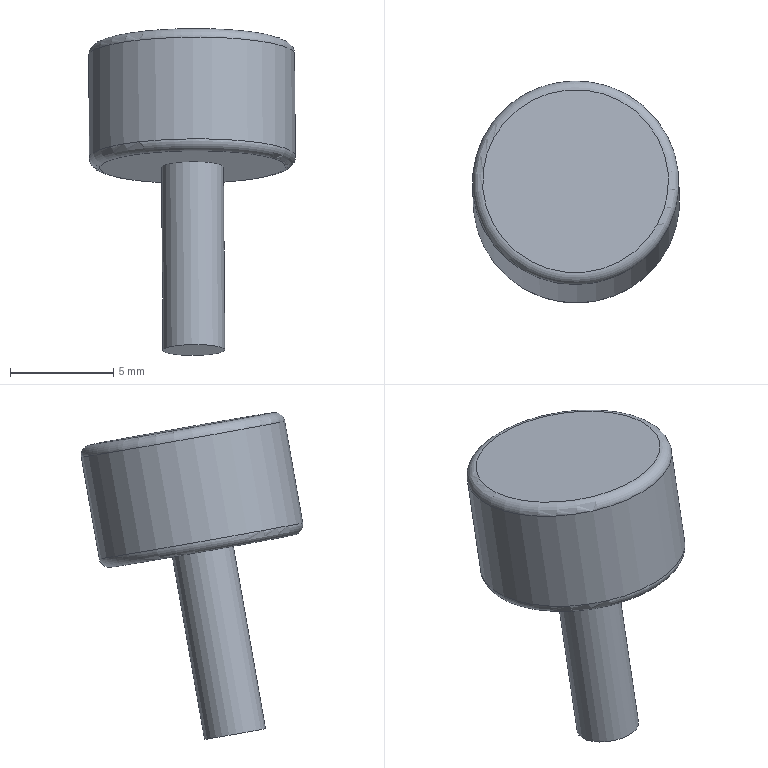Component | NX | 16 | 1 solid | 7 faces | box 10.04 x 10.73 x 15.82 mm | volume 532 mm3 | plane 3 | cylinder 2 | torus 2 | commonest cylinder face diameters 10 x1 3 x1
STEP:
#1=CARTESIAN_POINT('',(0.,0.,0.));
#2=DIRECTION('',(0.,0.,1.));
#3=DIRECTION('',(1.,0.,0.));
#4=AXIS2_PLACEMENT_3D('',#1,#2,#3);
#5=CARTESIAN_POINT('',(88.843,266.854,149.684));
#6=VERTEX_POINT('',#5);
#7=CARTESIAN_POINT('',(84.048,265.455,149.893));
#8=DIRECTION('',(0.00764,-0.1736,-0.9848));
#9=DIRECTION('',(0.9591,0.2798,-0.0419));
#10=AXIS2_PLACEMENT_3D('',#7,#8,#9);
#11=CIRCLE('',#10,5.);
#12=CARTESIAN_POINT('',(84.09,264.5,144.477));
#13=DIRECTION('',(-0.00764,0.1736,0.9848));
#14=DIRECTION('',(-0.9591,-0.2798,0.0419));
#15=AXIS2_PLACEMENT_3D('',#12,#13,#14);
#16=CYLINDRICAL_SURFACE('',#15,5.);
#17=CARTESIAN_POINT('',(9.425,5.5));
#18=DIRECTION('',(-1.,0.));
#19=VECTOR('',#18,1.);
#20=LINE('',#17,#19);
#21=(GEOMETRIC_REPRESENTATION_CONTEXT(2)PARAMETRIC_REPRESENTATION_CONTEXT()REPRESENTATION_CONTEXT('',''));
#22=DEFINITIONAL_REPRESENTATION('',(#20),#21);
#23=PCURVE('',#16,#22);
#24=CARTESIAN_POINT('',(84.048,265.455,149.893));
#25=DIRECTION('',(0.00764,-0.1736,-0.9848));
#26=DIRECTION('',(0.9591,0.2798,-0.0419));
#27=AXIS2_PLACEMENT_3D('',#24,#25,#26);
#28=TOROIDAL_SURFACE('',#27,4.5,0.5);
#29=CARTESIAN_POINT('',(0.,6.283));
#30=DIRECTION('',(1.,0.));
#31=VECTOR('',#30,1.);
#32=LINE('',#29,#31);
#33=(GEOMETRIC_REPRESENTATION_CONTEXT(2)PARAMETRIC_REPRESENTATION_CONTEXT()REPRESENTATION_CONTEXT('',''));
#34=DEFINITIONAL_REPRESENTATION('',(#32),#33);
#35=PCURVE('',#28,#34);
#36=SURFACE_CURVE('',#11,(#23,#35),.PCURVE_S1.);
#37=EDGE_CURVE('',#6,#6,#36,.T.);
#38=ORIENTED_EDGE('',*,*,#37,.T.);
#39=CARTESIAN_POINT('',(88.882,265.986,144.76));
#40=VERTEX_POINT('',#39);
#41=CARTESIAN_POINT('',(88.882,265.986,144.76));
#42=CARTESIAN_POINT('',(88.843,266.854,149.684));
#43=B_SPLINE_CURVE_WITH_KNOTS('',1,(#41,#42),.UNSPECIFIED.,.F.,.F.,(2,2),(0.5,5.5),.PIECEWISE_BEZIER_KNOTS.);
#44=CARTESIAN_POINT('',(3.142,0.));
#45=DIRECTION('',(0.,1.));
#46=VECTOR('',#45,1.);
#47=LINE('',#44,#46);
#48=(GEOMETRIC_REPRESENTATION_CONTEXT(2)PARAMETRIC_REPRESENTATION_CONTEXT()REPRESENTATION_CONTEXT('',''));
#49=DEFINITIONAL_REPRESENTATION('',(#47),#48);
#50=PCURVE('',#16,#49);
#51=CARTESIAN_POINT('',(9.425,0.));
#52=DIRECTION('',(0.,1.));
#53=VECTOR('',#52,1.);
#54=LINE('',#51,#53);
#55=(GEOMETRIC_REPRESENTATION_CONTEXT(2)PARAMETRIC_REPRESENTATION_CONTEXT()REPRESENTATION_CONTEXT('',''));
#56=DEFINITIONAL_REPRESENTATION('',(#54),#55);
#57=PCURVE('',#16,#56);
#58=SEAM_CURVE('',#43,(#50,#57),.PCURVE_S1.);
#59=EDGE_CURVE('',#40,#6,#58,.T.);
#60=ORIENTED_EDGE('',*,*,#59,.F.);
#61=CARTESIAN_POINT('',(84.086,264.586,144.969));
#62=DIRECTION('',(-0.00764,0.1736,0.9848));
#63=DIRECTION('',(0.9591,0.2798,-0.0419));
#64=AXIS2_PLACEMENT_3D('',#61,#62,#63);
#65=CIRCLE('',#64,5.);
#66=CARTESIAN_POINT('',(3.142,0.5));
#67=DIRECTION('',(1.,0.));
#68=VECTOR('',#67,1.);
#69=LINE('',#66,#68);
#70=(GEOMETRIC_REPRESENTATION_CONTEXT(2)PARAMETRIC_REPRESENTATION_CONTEXT()REPRESENTATION_CONTEXT('',''));
#71=DEFINITIONAL_REPRESENTATION('',(#69),#70);
#72=PCURVE('',#16,#71);
#73=CARTESIAN_POINT('',(84.086,264.586,144.969));
#74=DIRECTION('',(0.00764,-0.1736,-0.9848));
#75=DIRECTION('',(0.9591,0.2798,-0.0419));
#76=AXIS2_PLACEMENT_3D('',#73,#74,#75);
#77=TOROIDAL_SURFACE('',#76,4.5,0.5);
#78=CARTESIAN_POINT('',(6.283,6.283));
#79=CARTESIAN_POINT('',(6.188,6.283));
#80=CARTESIAN_POINT('',(5.998,6.283));
#81=CARTESIAN_POINT('',(5.712,6.283));
#82=CARTESIAN_POINT('',(5.426,6.283));
#83=CARTESIAN_POINT('',(5.141,6.283));
#84=CARTESIAN_POINT('',(4.855,6.283));
#85=CARTESIAN_POINT('',(4.57,6.283));
#86=CARTESIAN_POINT('',(4.284,6.283));
#87=CARTESIAN_POINT('',(3.998,6.283));
#88=CARTESIAN_POINT('',(3.713,6.283));
#89=CARTESIAN_POINT('',(3.427,6.283));
#90=CARTESIAN_POINT('',(3.142,6.283));
#91=CARTESIAN_POINT('',(2.856,6.283));
#92=CARTESIAN_POINT('',(2.57,6.283));
#93=CARTESIAN_POINT('',(2.285,6.283));
#94=CARTESIAN_POINT('',(1.999,6.283));
#95=CARTESIAN_POINT('',(1.714,6.283));
#96=CARTESIAN_POINT('',(1.428,6.283));
#97=CARTESIAN_POINT('',(1.142,6.283));
#98=CARTESIAN_POINT('',(0.8568,6.283));
#99=CARTESIAN_POINT('',(0.5712,6.283));
#100=CARTESIAN_POINT('',(0.2856,6.283));
#101=CARTESIAN_POINT('',(0.0952,6.283));
#102=CARTESIAN_POINT('',(0.,6.283));
#103=B_SPLINE_CURVE_WITH_KNOTS('',3,(#78,#79,#80,#81,#82,#83,#84,#85,#86,#87,#88,#89,#90,#91,#92,#93,#94,#95,#96,#97,#98,#99,#100,#101,#102),.UNSPECIFIED.,.F.,.F.,(4,1,1,1,1,1,1,1,1,1,1,1,1,1,1,1,1,1,1,1,1,1,4),(0.,0.2856,0.5712,0.8568,1.142,1.428,1.714,1.999,2.285,2.57,2.856,3.142,3.427,3.713,3.998,4.284,4.57,4.855,5.141,5.426,5.712,5.998,6.283),.QUASI_UNIFORM_KNOTS.);
#104=(GEOMETRIC_REPRESENTATION_CONTEXT(2)PARAMETRIC_REPRESENTATION_CONTEXT()REPRESENTATION_CONTEXT('',''));
#105=DEFINITIONAL_REPRESENTATION('',(#103),#104);
#106=PCURVE('',#77,#105);
#107=SURFACE_CURVE('',#65,(#72,#106),.PCURVE_S1.);
#108=EDGE_CURVE('',#40,#40,#107,.T.);
#109=ORIENTED_EDGE('',*,*,#108,.T.);
#110=ORIENTED_EDGE('',*,*,#59,.T.);
#111=EDGE_LOOP('',(#38,#60,#109,#110));
#112=FACE_BOUND('',#111,.T.);
#113=ADVANCED_FACE('',(#112),#16,.T.);
#114=CARTESIAN_POINT('',(88.406,265.759,144.288));
#115=VERTEX_POINT('',#114);
#116=CARTESIAN_POINT('',(84.09,264.5,144.477));
#117=DIRECTION('',(0.00764,-0.1736,-0.9848));
#118=DIRECTION('',(0.9591,0.2798,-0.0419));
#119=AXIS2_PLACEMENT_3D('',#116,#117,#118);
#120=CIRCLE('',#119,4.5);
#121=CARTESIAN_POINT('',(84.09,264.5,144.477));
#122=DIRECTION('',(0.00764,-0.1736,-0.9848));
#123=DIRECTION('',(0.9591,0.2798,-0.0419));
#124=AXIS2_PLACEMENT_3D('',#121,#122,#123);
#125=PLANE('',#124);
#126=CARTESIAN_POINT('',(0.,0.));
#127=DIRECTION('',(1.,0.));
#128=AXIS2_PLACEMENT_2D('',#126,#127);
#129=CIRCLE('',#128,4.5);
#130=(GEOMETRIC_REPRESENTATION_CONTEXT(2)PARAMETRIC_REPRESENTATION_CONTEXT()REPRESENTATION_CONTEXT('',''));
#131=DEFINITIONAL_REPRESENTATION('',(#129),#130);
#132=PCURVE('',#125,#131);
#133=CARTESIAN_POINT('',(0.,7.854));
#134=DIRECTION('',(1.,0.));
#135=VECTOR('',#134,1.);
#136=LINE('',#133,#135);
#137=(GEOMETRIC_REPRESENTATION_CONTEXT(2)PARAMETRIC_REPRESENTATION_CONTEXT()REPRESENTATION_CONTEXT('',''));
#138=DEFINITIONAL_REPRESENTATION('',(#136),#137);
#139=PCURVE('',#77,#138);
#140=SURFACE_CURVE('',#120,(#132,#139),.PCURVE_S1.);
#141=EDGE_CURVE('',#115,#115,#140,.T.);
#142=ORIENTED_EDGE('',*,*,#141,.T.);
#143=EDGE_LOOP('',(#142));
#144=FACE_BOUND('',#143,.T.);
#145=CARTESIAN_POINT('',(85.528,264.919,144.414));
#146=VERTEX_POINT('',#145);
#147=CARTESIAN_POINT('',(84.09,264.5,144.477));
#148=DIRECTION('',(0.00764,-0.1736,-0.9848));
#149=DIRECTION('',(0.9591,0.2798,-0.0419));
#150=AXIS2_PLACEMENT_3D('',#147,#148,#149);
#151=CIRCLE('',#150,1.5);
#152=CARTESIAN_POINT('',(0.,0.));
#153=DIRECTION('',(1.,-0.));
#154=AXIS2_PLACEMENT_2D('',#152,#153);
#155=CIRCLE('',#154,1.5);
#156=(GEOMETRIC_REPRESENTATION_CONTEXT(2)PARAMETRIC_REPRESENTATION_CONTEXT()REPRESENTATION_CONTEXT('',''));
#157=DEFINITIONAL_REPRESENTATION('',(#155),#156);
#158=PCURVE('',#125,#157);
#159=CARTESIAN_POINT('',(84.159,262.937,135.614));
#160=DIRECTION('',(-0.00764,0.1736,0.9848));
#161=DIRECTION('',(-0.9591,-0.2798,0.0419));
#162=AXIS2_PLACEMENT_3D('',#159,#160,#161);
#163=CYLINDRICAL_SURFACE('',#162,1.5);
#164=CARTESIAN_POINT('',(9.425,9.));
#165=DIRECTION('',(-1.,0.));
#166=VECTOR('',#165,1.);
#167=LINE('',#164,#166);
#168=(GEOMETRIC_REPRESENTATION_CONTEXT(2)PARAMETRIC_REPRESENTATION_CONTEXT()REPRESENTATION_CONTEXT('',''));
#169=DEFINITIONAL_REPRESENTATION('',(#167),#168);
#170=PCURVE('',#163,#169);
#171=SURFACE_CURVE('',#151,(#158,#170),.PCURVE_S1.);
#172=EDGE_CURVE('',#146,#146,#171,.T.);
#173=ORIENTED_EDGE('',*,*,#172,.F.);
#174=EDGE_LOOP('',(#173));
#175=FACE_BOUND('',#174,.T.);
#176=ADVANCED_FACE('',(#144,#175),#125,.T.);
#177=CARTESIAN_POINT('',(88.36,266.801,150.197));
#178=VERTEX_POINT('',#177);
#179=CARTESIAN_POINT('',(84.044,265.542,150.385));
#180=DIRECTION('',(-0.00764,0.1736,0.9848));
#181=DIRECTION('',(0.9591,0.2798,-0.0419));
#182=AXIS2_PLACEMENT_3D('',#179,#180,#181);
#183=CIRCLE('',#182,4.5);
#184=CARTESIAN_POINT('',(84.044,265.542,150.385));
#185=DIRECTION('',(0.00764,-0.1736,-0.9848));
#186=DIRECTION('',(0.9591,0.2798,-0.0419));
#187=AXIS2_PLACEMENT_3D('',#184,#185,#186);
#188=PLANE('',#187);
#189=CARTESIAN_POINT('',(4.5,0.));
#190=CARTESIAN_POINT('',(4.5,-7.794));
#191=CARTESIAN_POINT('',(-2.25,-3.897));
#192=CARTESIAN_POINT('',(-9.,-0.));
#193=CARTESIAN_POINT('',(-2.25,3.897));
#194=CARTESIAN_POINT('',(4.5,7.794));
#195=CARTESIAN_POINT('',(4.5,0.));
#196=(BOUNDED_CURVE()B_SPLINE_CURVE(2,(#189,#190,#191,#192,#193,#194,#195),.UNSPECIFIED.,.T.,.F.)B_SPLINE_CURVE_WITH_KNOTS((1,2,2,2,2,1),(-2.094,0.,2.094,4.189,6.283,8.378),.UNSPECIFIED.)CURVE()GEOMETRIC_REPRESENTATION_ITEM()RATIONAL_B_SPLINE_CURVE((1.,0.5,1.,0.5,1.,0.5,1.))REPRESENTATION_ITEM(''));
#197=(GEOMETRIC_REPRESENTATION_CONTEXT(2)PARAMETRIC_REPRESENTATION_CONTEXT()REPRESENTATION_CONTEXT('',''));
#198=DEFINITIONAL_REPRESENTATION('',(#196),#197);
#199=PCURVE('',#188,#198);
#200=CARTESIAN_POINT('',(6.283,4.712));
#201=DIRECTION('',(-1.,0.));
#202=VECTOR('',#201,1.);
#203=LINE('',#200,#202);
#204=(GEOMETRIC_REPRESENTATION_CONTEXT(2)PARAMETRIC_REPRESENTATION_CONTEXT()REPRESENTATION_CONTEXT('',''));
#205=DEFINITIONAL_REPRESENTATION('',(#203),#204);
#206=PCURVE('',#28,#205);
#207=SURFACE_CURVE('',#183,(#199,#206),.PCURVE_S1.);
#208=EDGE_CURVE('',#178,#178,#207,.T.);
#209=ORIENTED_EDGE('',*,*,#208,.T.);
#210=EDGE_LOOP('',(#209));
#211=FACE_BOUND('',#210,.T.);
#212=ADVANCED_FACE('',(#211),#188,.F.);
#213=CARTESIAN_POINT('',(85.597,263.357,135.551));
#214=VERTEX_POINT('',#213);
#215=CARTESIAN_POINT('',(84.159,262.937,135.614));
#216=DIRECTION('',(0.00764,-0.1736,-0.9848));
#217=DIRECTION('',(0.9591,0.2798,-0.0419));
#218=AXIS2_PLACEMENT_3D('',#215,#216,#217);
#219=CIRCLE('',#218,1.5);
#220=CARTESIAN_POINT('',(9.425,0.));
#221=DIRECTION('',(-1.,0.));
#222=VECTOR('',#221,1.);
#223=LINE('',#220,#222);
#224=(GEOMETRIC_REPRESENTATION_CONTEXT(2)PARAMETRIC_REPRESENTATION_CONTEXT()REPRESENTATION_CONTEXT('',''));
#225=DEFINITIONAL_REPRESENTATION('',(#223),#224);
#226=PCURVE('',#163,#225);
#227=CARTESIAN_POINT('',(84.159,262.937,135.614));
#228=DIRECTION('',(0.00764,-0.1736,-0.9848));
#229=DIRECTION('',(0.9591,0.2798,-0.0419));
#230=AXIS2_PLACEMENT_3D('',#227,#228,#229);
#231=PLANE('',#230);
#232=CARTESIAN_POINT('',(0.,0.));
#233=DIRECTION('',(1.,-0.));
#234=AXIS2_PLACEMENT_2D('',#232,#233);
#235=CIRCLE('',#234,1.5);
#236=(GEOMETRIC_REPRESENTATION_CONTEXT(2)PARAMETRIC_REPRESENTATION_CONTEXT()REPRESENTATION_CONTEXT('',''));
#237=DEFINITIONAL_REPRESENTATION('',(#235),#236);
#238=PCURVE('',#231,#237);
#239=SURFACE_CURVE('',#219,(#226,#238),.PCURVE_S1.);
#240=EDGE_CURVE('',#214,#214,#239,.T.);
#241=ORIENTED_EDGE('',*,*,#240,.F.);
#242=CARTESIAN_POINT('',(85.597,263.357,135.551));
#243=CARTESIAN_POINT('',(85.528,264.919,144.414));
#244=B_SPLINE_CURVE_WITH_KNOTS('',1,(#242,#243),.UNSPECIFIED.,.F.,.F.,(2,2),(0.,9.),.PIECEWISE_BEZIER_KNOTS.);
#245=CARTESIAN_POINT('',(9.425,0.));
#246=DIRECTION('',(0.,1.));
#247=VECTOR('',#246,1.);
#248=LINE('',#245,#247);
#249=(GEOMETRIC_REPRESENTATION_CONTEXT(2)PARAMETRIC_REPRESENTATION_CONTEXT()REPRESENTATION_CONTEXT('',''));
#250=DEFINITIONAL_REPRESENTATION('',(#248),#249);
#251=PCURVE('',#163,#250);
#252=CARTESIAN_POINT('',(3.142,0.));
#253=DIRECTION('',(0.,1.));
#254=VECTOR('',#253,1.);
#255=LINE('',#252,#254);
#256=(GEOMETRIC_REPRESENTATION_CONTEXT(2)PARAMETRIC_REPRESENTATION_CONTEXT()REPRESENTATION_CONTEXT('',''));
#257=DEFINITIONAL_REPRESENTATION('',(#255),#256);
#258=PCURVE('',#163,#257);
#259=SEAM_CURVE('',#244,(#251,#258),.PCURVE_S1.);
#260=EDGE_CURVE('',#214,#146,#259,.T.);
#261=ORIENTED_EDGE('',*,*,#260,.T.);
#262=ORIENTED_EDGE('',*,*,#172,.T.);
#263=ORIENTED_EDGE('',*,*,#260,.F.);
#264=EDGE_LOOP('',(#241,#261,#262,#263));
#265=FACE_BOUND('',#264,.T.);
#266=ADVANCED_FACE('',(#265),#163,.T.);
#267=ORIENTED_EDGE('',*,*,#240,.T.);
#268=EDGE_LOOP('',(#267));
#269=FACE_BOUND('',#268,.T.);
#270=ADVANCED_FACE('',(#269),#231,.T.);
#271=ORIENTED_EDGE('',*,*,#208,.F.);
#272=CARTESIAN_POINT('',(88.36,266.801,150.197));
#273=CARTESIAN_POINT('',(88.488,266.838,150.191));
#274=CARTESIAN_POINT('',(88.613,266.867,150.144));
#275=CARTESIAN_POINT('',(88.722,266.884,150.059));
#276=CARTESIAN_POINT('',(88.801,266.888,149.945));
#277=CARTESIAN_POINT('',(88.842,266.877,149.815));
#278=CARTESIAN_POINT('',(88.843,266.854,149.684));
#279=(BOUNDED_CURVE()B_SPLINE_CURVE(6,(#272,#273,#274,#275,#276,#277,#278),.UNSPECIFIED.,.F.,.F.)B_SPLINE_CURVE_WITH_KNOTS((7,7),(4.712,6.283),.PIECEWISE_BEZIER_KNOTS.)CURVE()GEOMETRIC_REPRESENTATION_ITEM()RATIONAL_B_SPLINE_CURVE((1.031,1.01,0.9979,0.994,0.9979,1.01,1.031))REPRESENTATION_ITEM(''));
#280=CARTESIAN_POINT('',(6.283,0.));
#281=DIRECTION('',(0.,1.));
#282=VECTOR('',#281,1.);
#283=LINE('',#280,#282);
#284=(GEOMETRIC_REPRESENTATION_CONTEXT(2)PARAMETRIC_REPRESENTATION_CONTEXT()REPRESENTATION_CONTEXT('',''));
#285=DEFINITIONAL_REPRESENTATION('',(#283),#284);
#286=PCURVE('',#28,#285);
#287=CARTESIAN_POINT('',(0.,0.));
#288=DIRECTION('',(0.,1.));
#289=VECTOR('',#288,1.);
#290=LINE('',#287,#289);
#291=(GEOMETRIC_REPRESENTATION_CONTEXT(2)PARAMETRIC_REPRESENTATION_CONTEXT()REPRESENTATION_CONTEXT('',''));
#292=DEFINITIONAL_REPRESENTATION('',(#290),#291);
#293=PCURVE('',#28,#292);
#294=SEAM_CURVE('',#279,(#286,#293),.PCURVE_S1.);
#295=EDGE_CURVE('',#178,#6,#294,.T.);
#296=ORIENTED_EDGE('',*,*,#295,.T.);
#297=ORIENTED_EDGE('',*,*,#37,.F.);
#298=ORIENTED_EDGE('',*,*,#295,.F.);
#299=EDGE_LOOP('',(#271,#296,#297,#298));
#300=FACE_BOUND('',#299,.T.);
#301=ADVANCED_FACE('',(#300),#28,.T.);
#302=ORIENTED_EDGE('',*,*,#108,.F.);
#303=CARTESIAN_POINT('',(88.882,265.986,144.76));
#304=CARTESIAN_POINT('',(88.883,265.962,144.628));
#305=CARTESIAN_POINT('',(88.843,265.928,144.502));
#306=CARTESIAN_POINT('',(88.766,265.886,144.395));
#307=CARTESIAN_POINT('',(88.659,265.84,144.319));
#308=CARTESIAN_POINT('',(88.534,265.796,144.283));
#309=CARTESIAN_POINT('',(88.406,265.759,144.288));
#310=(BOUNDED_CURVE()B_SPLINE_CURVE(6,(#303,#304,#305,#306,#307,#308,#309),.UNSPECIFIED.,.F.,.F.)B_SPLINE_CURVE_WITH_KNOTS((7,7),(6.283,7.854),.PIECEWISE_BEZIER_KNOTS.)CURVE()GEOMETRIC_REPRESENTATION_ITEM()RATIONAL_B_SPLINE_CURVE((1.031,1.01,0.9979,0.994,0.9979,1.01,1.031))REPRESENTATION_ITEM(''));
#311=CARTESIAN_POINT('',(6.283,0.));
#312=DIRECTION('',(0.,1.));
#313=VECTOR('',#312,1.);
#314=LINE('',#311,#313);
#315=(GEOMETRIC_REPRESENTATION_CONTEXT(2)PARAMETRIC_REPRESENTATION_CONTEXT()REPRESENTATION_CONTEXT('',''));
#316=DEFINITIONAL_REPRESENTATION('',(#314),#315);
#317=PCURVE('',#77,#316);
#318=CARTESIAN_POINT('',(0.,0.));
#319=DIRECTION('',(0.,1.));
#320=VECTOR('',#319,1.);
#321=LINE('',#318,#320);
#322=(GEOMETRIC_REPRESENTATION_CONTEXT(2)PARAMETRIC_REPRESENTATION_CONTEXT()REPRESENTATION_CONTEXT('',''));
#323=DEFINITIONAL_REPRESENTATION('',(#321),#322);
#324=PCURVE('',#77,#323);
#325=SEAM_CURVE('',#310,(#317,#324),.PCURVE_S1.);
#326=EDGE_CURVE('',#40,#115,#325,.T.);
#327=ORIENTED_EDGE('',*,*,#326,.T.);
#328=ORIENTED_EDGE('',*,*,#141,.F.);
#329=ORIENTED_EDGE('',*,*,#326,.F.);
#330=EDGE_LOOP('',(#302,#327,#328,#329));
#331=FACE_BOUND('',#330,.T.);
#332=ADVANCED_FACE('',(#331),#77,.T.);
#333=CLOSED_SHELL('',(#113,#176,#212,#266,#270,#301,#332));
#334=MANIFOLD_SOLID_BREP('',#333);
#335=(LENGTH_UNIT()NAMED_UNIT(*)SI_UNIT(.MILLI.,.METRE.));
#336=UNCERTAINTY_MEASURE_WITH_UNIT(LENGTH_MEASURE(0.00001),#335,'','');
#337=(NAMED_UNIT(*)PLANE_ANGLE_UNIT()SI_UNIT($,.RADIAN.));
#338=(NAMED_UNIT(*)SI_UNIT($,.STERADIAN.)SOLID_ANGLE_UNIT());
#339=(GEOMETRIC_REPRESENTATION_CONTEXT(3)GLOBAL_UNCERTAINTY_ASSIGNED_CONTEXT((#336))GLOBAL_UNIT_ASSIGNED_CONTEXT((#335,#337,#338))REPRESENTATION_CONTEXT('',''));
#340=ADVANCED_BREP_SHAPE_REPRESENTATION('',(#4,#334),#339);